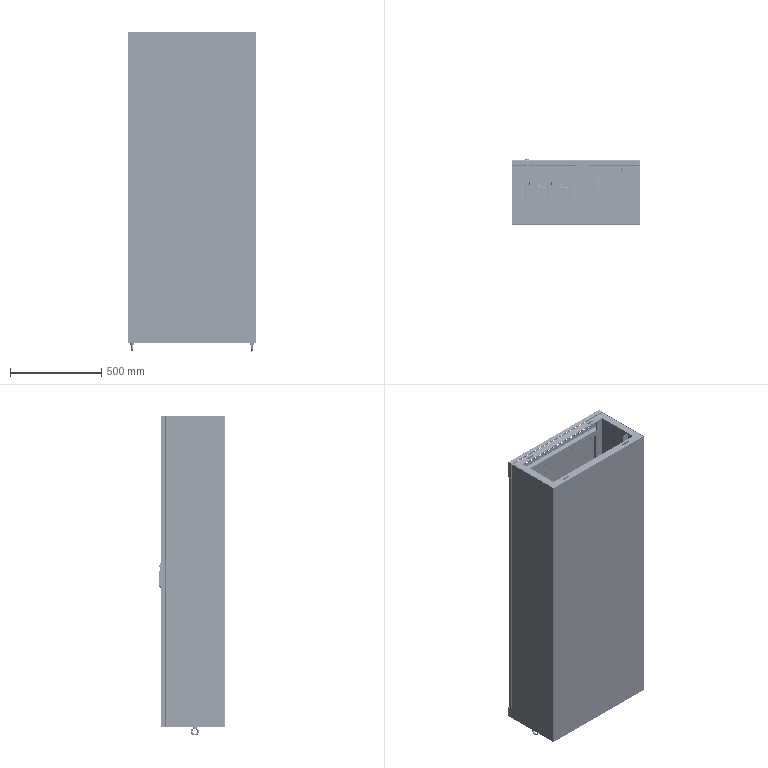Assembly | SolidWorks | mm | 157 component files | 161 solids | 10150 faces | box 700 x 358.26 x 1744.89 mm | volume 31550326 mm3 | plane 7176 | cylinder 2560 | cone 364 | torus 40 | sphere 10 | commonest cylinder face diameters 7 x828 9 x406 4.2 x320 5 x305 6 x156 10 x88 1 x74 3 x44
Bill of materials:
CabinetDepthBeam | 2 |  | Straight equal-leg-looking L-section (angle) bar with a small inside bend radius and plain square-cut ends; no holes visible.
CabinetWidthBeam | 2 |  | Long L-section (angle) strip with a rounded bend. One flange has two elongated slots near its ends, and that flange is trimmed short at both ends, so the other flange sticks out past it.
Brow | 1 |  | Long, slender, thin-walled channel or box-like rail with a top flange, a back web and a lower lip or flange. The lower edge has two small rectangular notches, one near each end.
BrowBracket | 2 |  | Short U- or C-shaped bent sheet bracket with rounded bends. Its web has one round through-hole in the middle, and the two parallel flanges are plain.
hexagon head bolts-full thread gb | 2 |  | Hex-head bolt-like fastener. It has a hexagonal head with a chamfered top, a bearing-face ring under the head, a plain cylindrical shank and a chamfered tip.
C120HighCurrentMiniatureCircuitBreaker | 8 |  | Compact stepped rectangular block with notches or recesses on one side, a square opening in the top face, small side features, and a rounded boss with a thin pin-like tab sticking out from one side.
CableSupportBracket | 2 |  | C-shaped (channel) bent sheet strip with two equal parallel flanges, a flat web and rounded bends; no holes visible.
Column | 2 |  | Long, slender L-section (angle) strip with a rounded bend. One face has a single row of many small, evenly spaced elongated slots along its length.
hex nuts, style 1-grades ab gb | 2 |  | Hexagonal nut-like part with a round central through-bore and chamfered corners on both faces.
HH54PIntermediateRelay | 6 |  | Solid stepped block made of a taller rectangular prism with a shorter rectangular prism attached to one side, giving an L or T silhouette.
HHL011-1RittalHinge | 2 |  | Hinge-leaf-like part: a thick flat leaf with three countersunk-looking through-holes in a row, and two cylindrical knuckles with axial bores on an offset arm, separated by a gap.
HHL011-1RittalHingePin | 4 |  | Headed cylindrical pin with a short, larger-diameter head that has a rounded edge, a plain shank, and a rounded or chamfered tip.
LC1-D40..D65(3-pole)ContactorSchneider | 6 |  | Compact prismatic block with multiple stepped faces, a raised ledge along one side, and small recesses on the top face.
LowerSill | 1 |  | Long thin formed sheet-metal-style channel with a stepped Z/hook-like cross-section and a row of many narrow vertical slots in the main web.
LRD340CThermalRelaySchneider | 4 |  | Stepped rectangular body with a chamfered upper edge, three square recesses on the top face, and three straight pins projecting from the bottom.
M12LiftingEye | 2 |  | Torus (ring of circular cross-section) truncated by a flat plane, leaving a two-lobed (figure-eight-like) planar face.
M12LiftingEyeInterruption | 2 |  | Threaded fastener with a short cylindrical head with chamfered edges and an externally threaded shank.
M12Nut | 2 |  | Hexagonal prism with a plain cylindrical through-bore, nut-like.
M6PhillipsSelf-tappingScrew | 4 |  | Pan/cheese-style head screw with a cross-shaped drive recess and a threaded shank.
MountingBeam | 6 |  | Long thin-walled C-channel with rows of obround slots along the web.
NSX100F-3PMoldedCase | 2 |  | Rectangular box-like body with three rectangular openings in the top, small round holes on one face, and a stepped projecting feature with a thin protruding blade/tab on one side.
HHL011-1RittalHingeMiddleShaftSleeve | 2 |  | Hinge-leaf-like bent strip: flat leaf with two round holes, an offset S-bend, and a rolled curl forming a segmented knuckle.
MMS480-2A-1Lock | 1 |  | Obround flanged plug/insert with a thin rim and a body cut by a C-shaped notch on one side.
OuterDoor1536X696 | 1 |  | Thin flat rectangular plate with one elongated slot and a pattern of small round holes near one end.
RightSidePanel | 1 |  | Long, straight thin-wall angle profile with two legs at roughly 90 degrees. Both leg edges end in short return lips, and one leg also has a short inward flange. The section is constant along the whole length.
SidePanel | 1 |  | Long, straight thin-wall angle profile, apparently the mirror image of a similar angle part. Two perpendicular legs, each with short return lips, and one leg with a short flange at its edge. The section is constant along the whole length.
TopCoverPlate | 1 |  | Bent thin-sheet bracket with a Z-shaped section: a large flat rectangular base plate, a vertical wall along one long edge, and a short flange at the top of the wall pointing outward. The base plate has two small round holes near its ends, and the wall has two more.
UK5NFuseTerminal | 4 |  | Thick flat plate with an irregular outline: chamfered corners on one side, a thin angled tab sticking out from one top corner, a stepped notch at the opposite top corner, and a wide rectangular recess along the bottom edge with undercut lips. One edge region steps down in thickness.
UK5NVoltageTerminalBlock | 80 |  | Thick flat plate with a roughly X- or hourglass-shaped outline: four splayed arms, short flats at the top corners, and a wide rectangular recess along the bottom edge with angled hook-like lips. A small pocket in one end face contains a small cylindrical pin-like feature.
VoltageTerminalRail | 1 |  | Long, slender hat-section (top-hat) profile: a central recessed channel with two flat side flanges and rounded bends. A continuous row of evenly spaced elongated slots runs along the length.
WATSGA-160A-4PCRDualPower | 1 |  | Rectangular box-shaped body with a larger flat flange plate on one face, which has four corner holes. Two rows of four flat rectangular tabs, each with a round hole, stick out from opposite sides of the body. An L-shaped lever handle sits on a stepped cylindrical shaft on the face opposite the flange. There is a small notch on one top edge.
Mates:
1. concentric | OuterDoorAssembly1-1/HHL011-1RittalHingeMiddleShaftSleeve-2 face at (542.975, 175.307, 245.51) dir (0, 0, -1) r 5.999 | HHL011-1RittalHinge-1 face at (542.975, 175.307, 190.51) dir (0, 0, 1) r 6
2. concentric | OuterDoorAssembly1-1/HHL011-1RittalHingeMiddleShaftSleeve-2 face at (542.975, 175.307, 245.51) dir (0, 0, -1) r 5.999 | HHL011-1RittalHinge-1 face at (542.975, 175.307, 190.51) dir (0, 0, 1) r 6
3. coincident | OuterDoorAssembly1-1/HHL011-1RittalHingeMiddleShaftSleeve-2 face at (535.132, 193.246, 210.51) dir (0, 0, -1) | HHL011-1RittalHinge-1 face at (524.475, 178.307, 210.51) dir (0, 0, 1)
4. lock | SidePanel-1 reference at (0, 0, 0) dir (1, 0, 0) | RightSidePanel-1 reference at (0, 0, 0) dir (1, 0, 0)
5. lock | SidePanel-1 reference at (0, 0, 0) dir (1, 0, 0) | TopCoverPlate-1 reference at (0, 0, 0) dir (1, 0, 0)
6. lock | RightSidePanel-1 reference at (0, 0, 0) dir (1, 0, 0) | LowerSill-1 reference at (0, 0, 0) dir (1, 0, 0)
7. lock | SidePanel-1 reference at (0, 0, 0) dir (1, 0, 0) | Brow-1 reference at (0, 0, 0) dir (1, 0, 0)
8. lock | Brow-1 reference at (0, 0, 0) dir (1, 0, 0) | BrowBracketAssembly3-1/BrowBracket-1 reference at (0, 0, 0) dir (1, 0, 0)
9. lock | TopCoverPlate-1 reference at (0, 0, 0) dir (1, 0, 0) | BrowBracketAssembly3-2/BrowBracket-1 reference at (0, 0, 0) dir (1, 0, 0)
10. lock | BrowBracketAssembly3-1/hexagon head bolts-full thread gb-2 reference at (0, 0, 0) dir (1, 0, 0) | hex nuts, style 1-grades ab gb-2 reference at (0, 0, 0) dir (1, 0, 0)
11. lock | BrowBracketAssembly3-2/hexagon head bolts-full thread gb-2 reference at (0, 0, 0) dir (1, 0, 0) | hex nuts, style 1-grades ab gb-1 reference at (0, 0, 0) dir (1, 0, 0)
12. lock | SidePanel-1 reference at (0, 0, 0) dir (1, 0, 0) | BottomFrameAssembly2-1/CabinetDepthBeam-2 reference at (0, 0, 0) dir (1, 0, 0)
13. lock | SidePanel-1 reference at (0, 0, 0) dir (1, 0, 0) | Column-8 reference at (0, 0, 0) dir (1, 0, 0)
14. lock | RightSidePanel-1 reference at (0, 0, 0) dir (1, 0, 0) | Column-4 reference at (0, 0, 0) dir (1, 0, 0)
15. lock | RightSidePanel-1 reference at (0, 0, 0) dir (1, 0, 0) | M6PhillipsSelf-tappingScrew-3 reference at (0, 0, 0) dir (1, 0, 0)
16. lock | RightSidePanel-1 reference at (0, 0, 0) dir (1, 0, 0) | M6PhillipsSelf-tappingScrew-4 reference at (0, 0, 0) dir (1, 0, 0)
17. lock | RightSidePanel-1 reference at (0, 0, 0) dir (1, 0, 0) | M6PhillipsSelf-tappingScrew-1 reference at (0, 0, 0) dir (1, 0, 0)
18. lock | RightSidePanel-1 reference at (0, 0, 0) dir (1, 0, 0) | M6PhillipsSelf-tappingScrew-2 reference at (0, 0, 0) dir (1, 0, 0)
19. lock | RightSidePanel-1 reference at (0, 0, 0) dir (1, 0, 0) | HHL011-1RittalHinge-1 reference at (0, 0, 0) dir (1, 0, 0)
20. lock | RightSidePanel-1 reference at (0, 0, 0) dir (1, 0, 0) | HHL011-1RittalHinge-2 reference at (0, 0, 0) dir (1, 0, 0)
21. lock | HHL011-1RittalHinge-2 reference at (0, 0, 0) dir (1, 0, 0) | HHL011-1RittalHingePin-3 reference at (0, 0, 0) dir (1, 0, 0)
22. lock | HHL011-1RittalHinge-2 reference at (0, 0, 0) dir (1, 0, 0) | HHL011-1RittalHingePin-2 reference at (0, 0, 0) dir (1, 0, 0)
23. lock | HHL011-1RittalHinge-1 reference at (0, 0, 0) dir (1, 0, 0) | HHL011-1RittalHingePin-4 reference at (0, 0, 0) dir (1, 0, 0)
24. lock | HHL011-1RittalHinge-1 reference at (0, 0, 0) dir (1, 0, 0) | HHL011-1RittalHingePin-1 reference at (0, 0, 0) dir (1, 0, 0)
25. lock | TopCoverPlate-1 reference at (0, 0, 0) dir (1, 0, 0) | M12LiftingEyeAssembly1-2/M12LiftingEye-1 reference at (0, 0, 0) dir (1, 0, 0)
26. lock | TopCoverPlate-1 reference at (0, 0, 0) dir (1, 0, 0) | M12LiftingEyeAssembly1-1/M12LiftingEye-1 reference at (0, 0, 0) dir (1, 0, 0)
27. lock | TopCoverPlate-1 reference at (0, 0, 0) dir (1, 0, 0) | M12Nut-2 reference at (0, 0, 0) dir (1, 0, 0)
28. lock | TopCoverPlate-1 reference at (0, 0, 0) dir (1, 0, 0) | M12Nut-1 reference at (0, 0, 0) dir (1, 0, 0)
29. lock | RightSidePanel-1 reference at (0, 0, 0) dir (1, 0, 0) | CableSupportBracket-1 reference at (0, 0, 0) dir (1, 0, 0)
30. lock | BrowBracket-1 reference at (0, 0, 0) dir (1, 0, 0) | hexagon head bolts-full thread gb-2 reference at (0, 0, 0) dir (1, 0, 0)
31. lock | M12LiftingEye-1 reference at (0, 0, 0) dir (1, 0, 0) | M12LiftingEyeInterruption-2 reference at (0, 0, 0) dir (1, 0, 0)
32. lock | OuterDoor1536X696-1 reference at (0, 0, 0) dir (1, 0, 0) | MMS480-2A-1Lock-1 reference at (0, 0, 0) dir (1, 0, 0)
33. lock | OuterDoor1536X696-1 reference at (0, 0, 0) dir (1, 0, 0) | CableSupportBracket-1 reference at (0, 0, 0) dir (1, 0, 0)